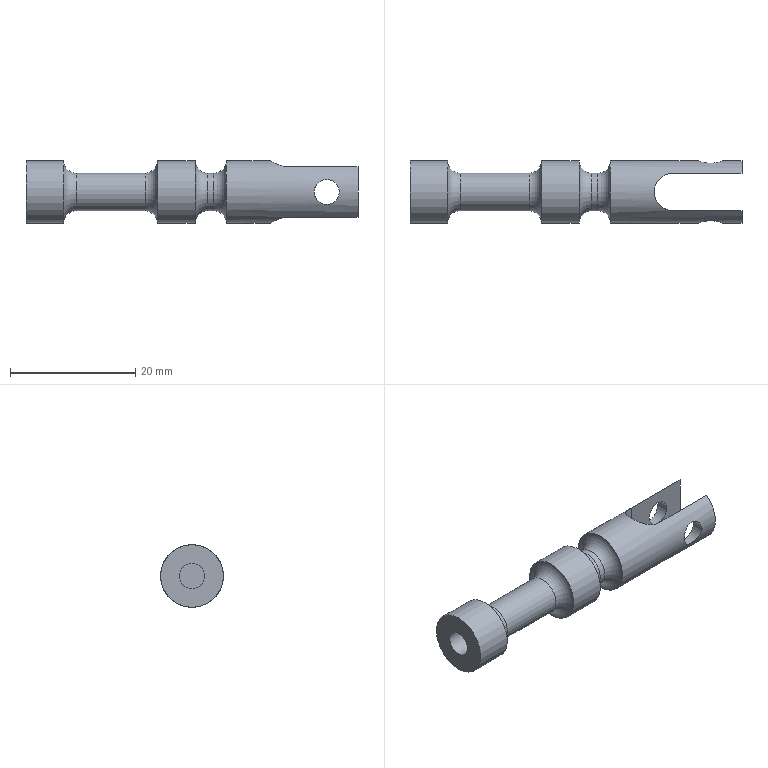Component | NX | EXTERNAL_PISTON | 1 solid | 19 faces | volume 2029 mm3 | cylinder 9 | plane 6 | torus 4 | commonest cylinder face diameters 10 x3 6 x3 4 x3